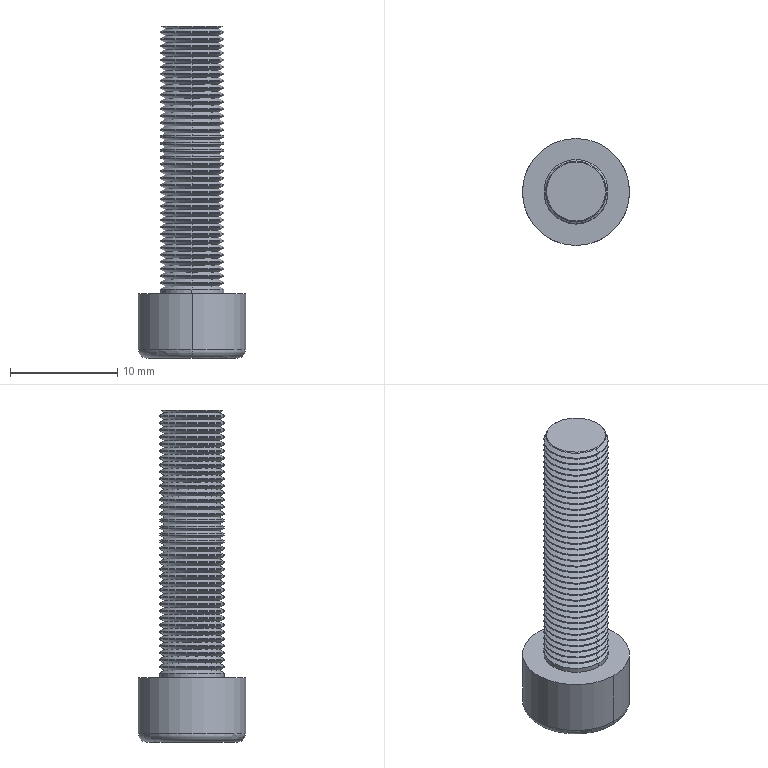Component | SolidWorks | LongSideClampingAssemblyBGeneralAssembly-1_HexagonSocketHeadCapScrew-M6X25-0510-2 | 1 solid | 251 faces | box 10 x 10 x 31 mm | volume 1014 mm3 | cone 156 | cylinder 78 | plane 15 | torus 2 | commonest cylinder face diameters 6 x76 10 x2
build123d program:
from build123d import *

# Parameters (mm, degrees)
SKETCH1_R           = 5
BASEHEAD_DEPTH      = 6
SKETCH2_R           = 3
BASEBODY_DEPTH      = 25
HEXAGONSOCKET_DEPTH = 3
TOPFILLET_R         = 0.75
CHAMFER1_SIZE       = 0.25
LPATTERN10_COUNT    = 38
LPATTERN10_PITCH    = 0.6498


with BuildPart() as part:
    # Sketch1 → BaseHead (new body)
    with BuildSketch(Plane(origin=(0, 0, 0), x_dir=(0, 0, -1), z_dir=(1, 0, 0))):
        Circle(SKETCH1_R)
    extrude(amount=BASEHEAD_DEPTH)

    # Sketch2 → BaseBody (add)
    with BuildSketch(Plane(origin=(6, 0, 0), x_dir=(0, 0, -1), z_dir=(1, 0, 0))):
        Circle(SKETCH2_R)
    extrude(amount=BASEBODY_DEPTH)

    # Sketch3 → HexagonSocket (cut)
    with BuildSketch(Plane(origin=(0, 0, 0), x_dir=(0, 0, -1), z_dir=(1, 0, 0))):
        Polygon((2.887, 0), (1.443, 2.5), (-1.443, 2.5), (-2.887, 0), (-1.443, -2.5), (1.443, -2.5), align=None)
    extrude(amount=HEXAGONSOCKET_DEPTH, mode=Mode.SUBTRACT)

    # Sketch4 → Cut-Revolve1 (revolve, cut)
    with BuildSketch(Plane(origin=(-4.196, 0.75, 0), x_dir=(-1, 0, 0), z_dir=(0, 0, 1)), mode=Mode.PRIVATE) as cut_revolve1_sk:
        Polygon((-7.196, 3.25), (-8.64, 0.75), (-7.196, 0.75), align=None)
    revolve(cut_revolve1_sk.sketch.rotate(Axis((0.839, 0, 0), (-1, 0, 0)), 90), axis=Axis((0.839, 0, 0), (-1, 0, 0)), mode=Mode.SUBTRACT)

    # TopFillet
    topfillet_edges = [part.edges().sort_by_distance(p)[0] for p in [
        (0, 0, 5),
    ]]
    fillet(topfillet_edges, radius=TOPFILLET_R)

    # Chamfer1
    chamfer1_edges = [part.edges().sort_by_distance(p)[0] for p in [
        (31, 0, 3),
    ]]
    chamfer(chamfer1_edges, length=CHAMFER1_SIZE)

    # Sketch5 → Cut-Revolve10 (revolve, cut)
    with BuildSketch(Plane.XY, mode=Mode.PRIVATE) as cut_revolve10_sk:
        Polygon((30.75, 2.531), (31.021, 3), (31.021, 3.542), (30.479, 3.542), (30.479, 3), align=None)
    cut_revolve10 = revolve(cut_revolve10_sk.sketch.rotate(Axis((0, 0, 0), (1, 0, 0)), 90), axis=Axis((0, 0, 0), (1, 0, 0)), mode=Mode.SUBTRACT)

    # LPattern10: Cut-Revolve10 ×38
    with Locations(*[(-i * LPATTERN10_PITCH, 0, 0) for i in range(1, LPATTERN10_COUNT)]):
        add(cut_revolve10, mode=Mode.SUBTRACT)


solid = part.part

# Placed as in the assembly
solid = solid.moved(Location((-3103.658, -50.609, 3487.3), (90, 0, 90)))